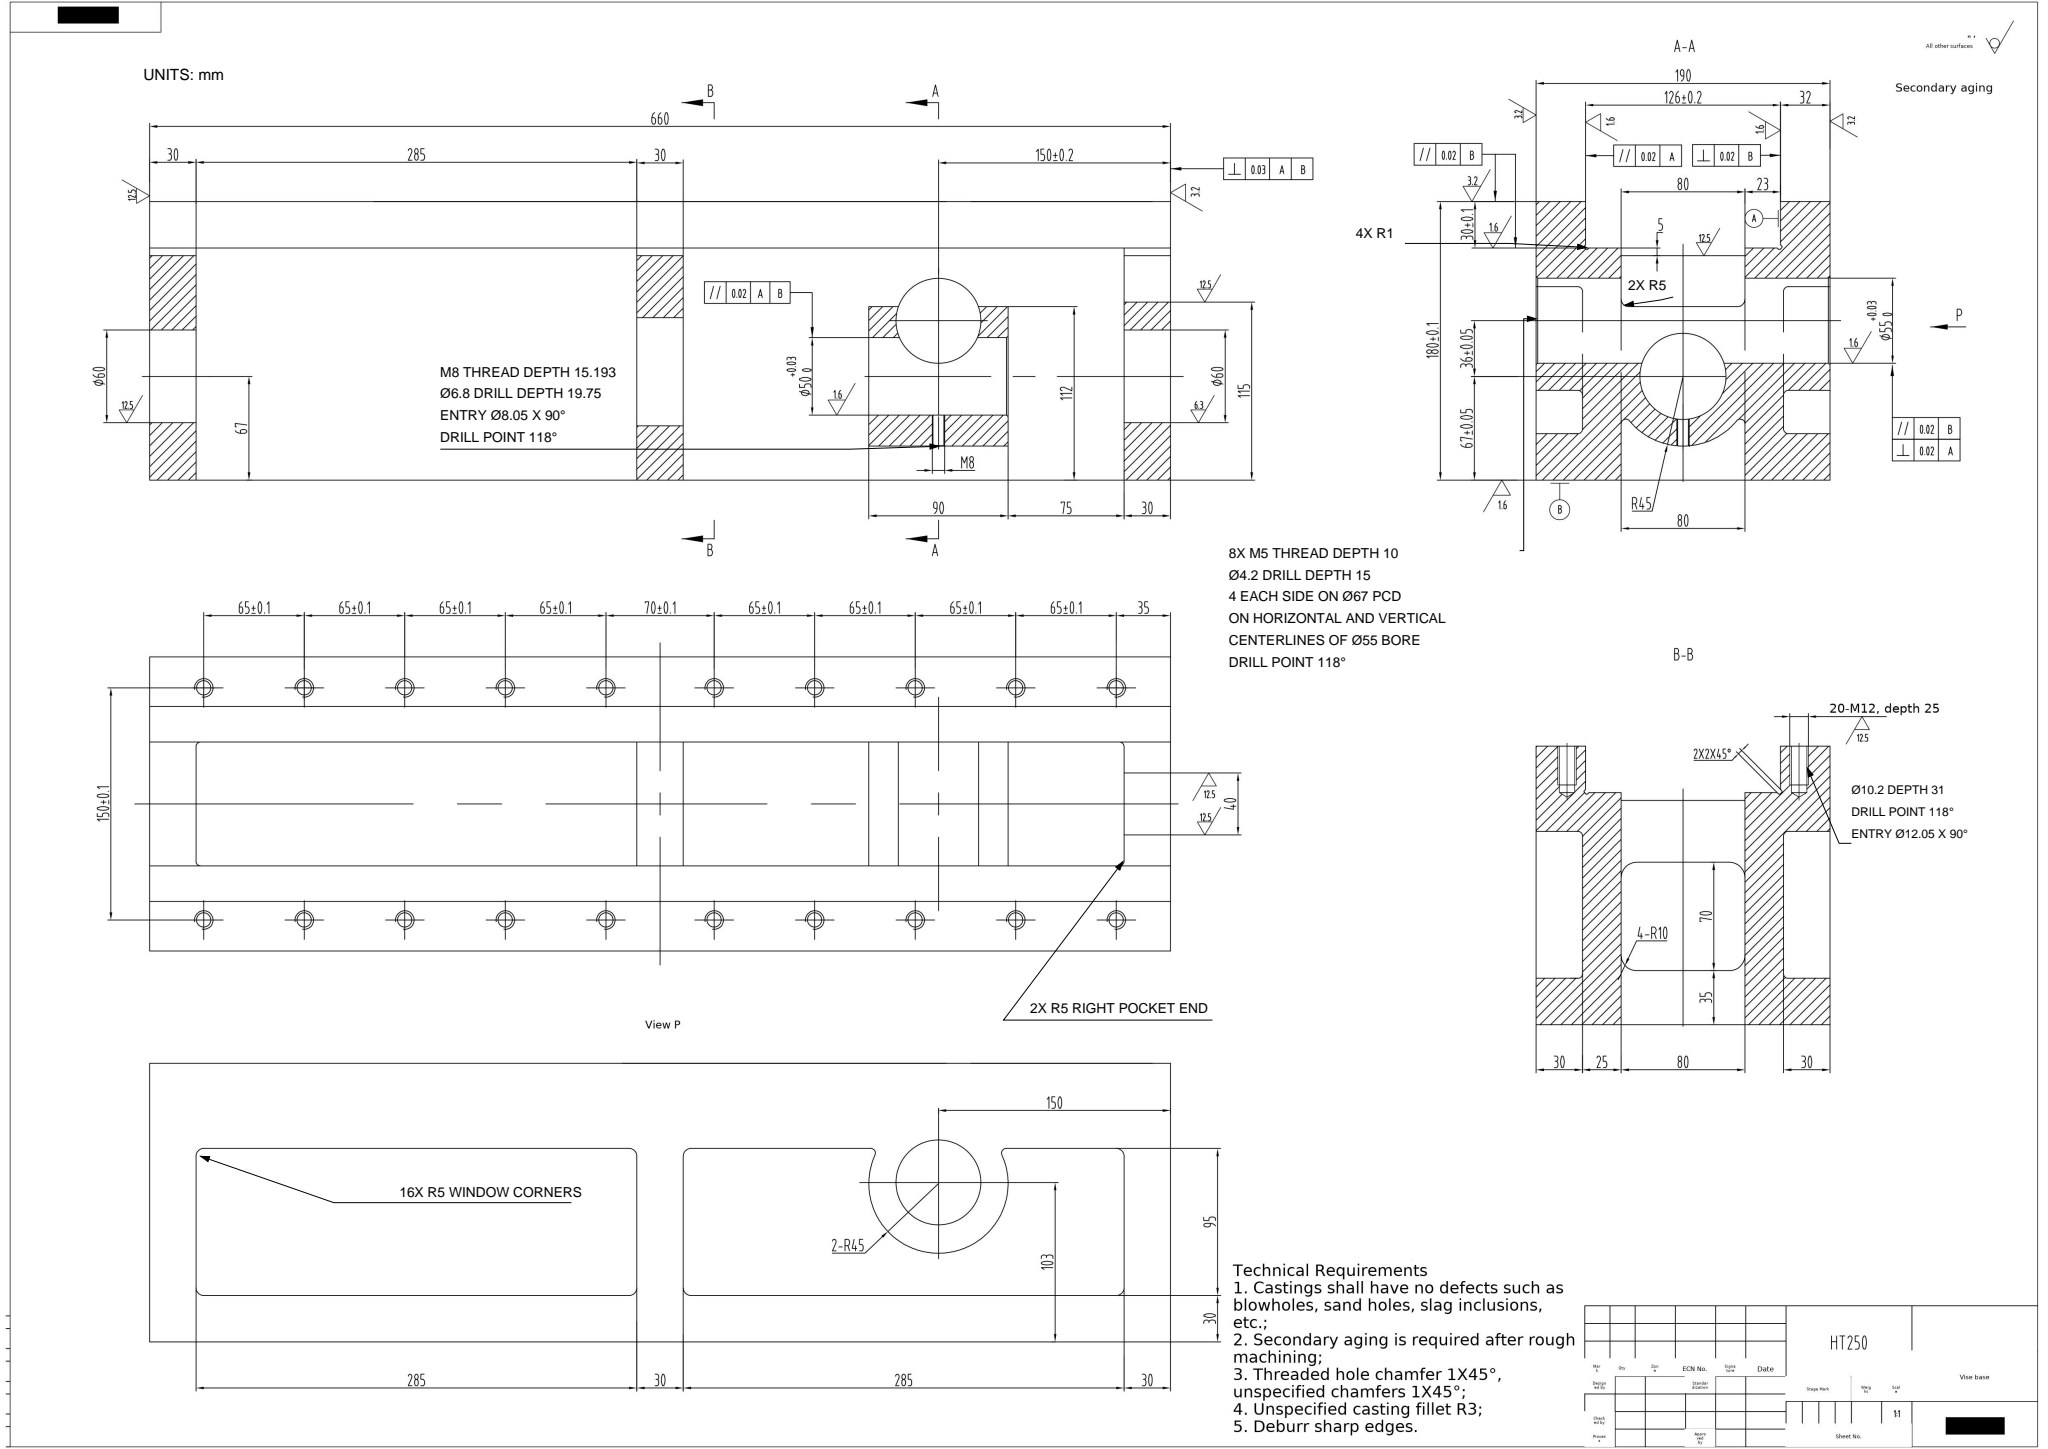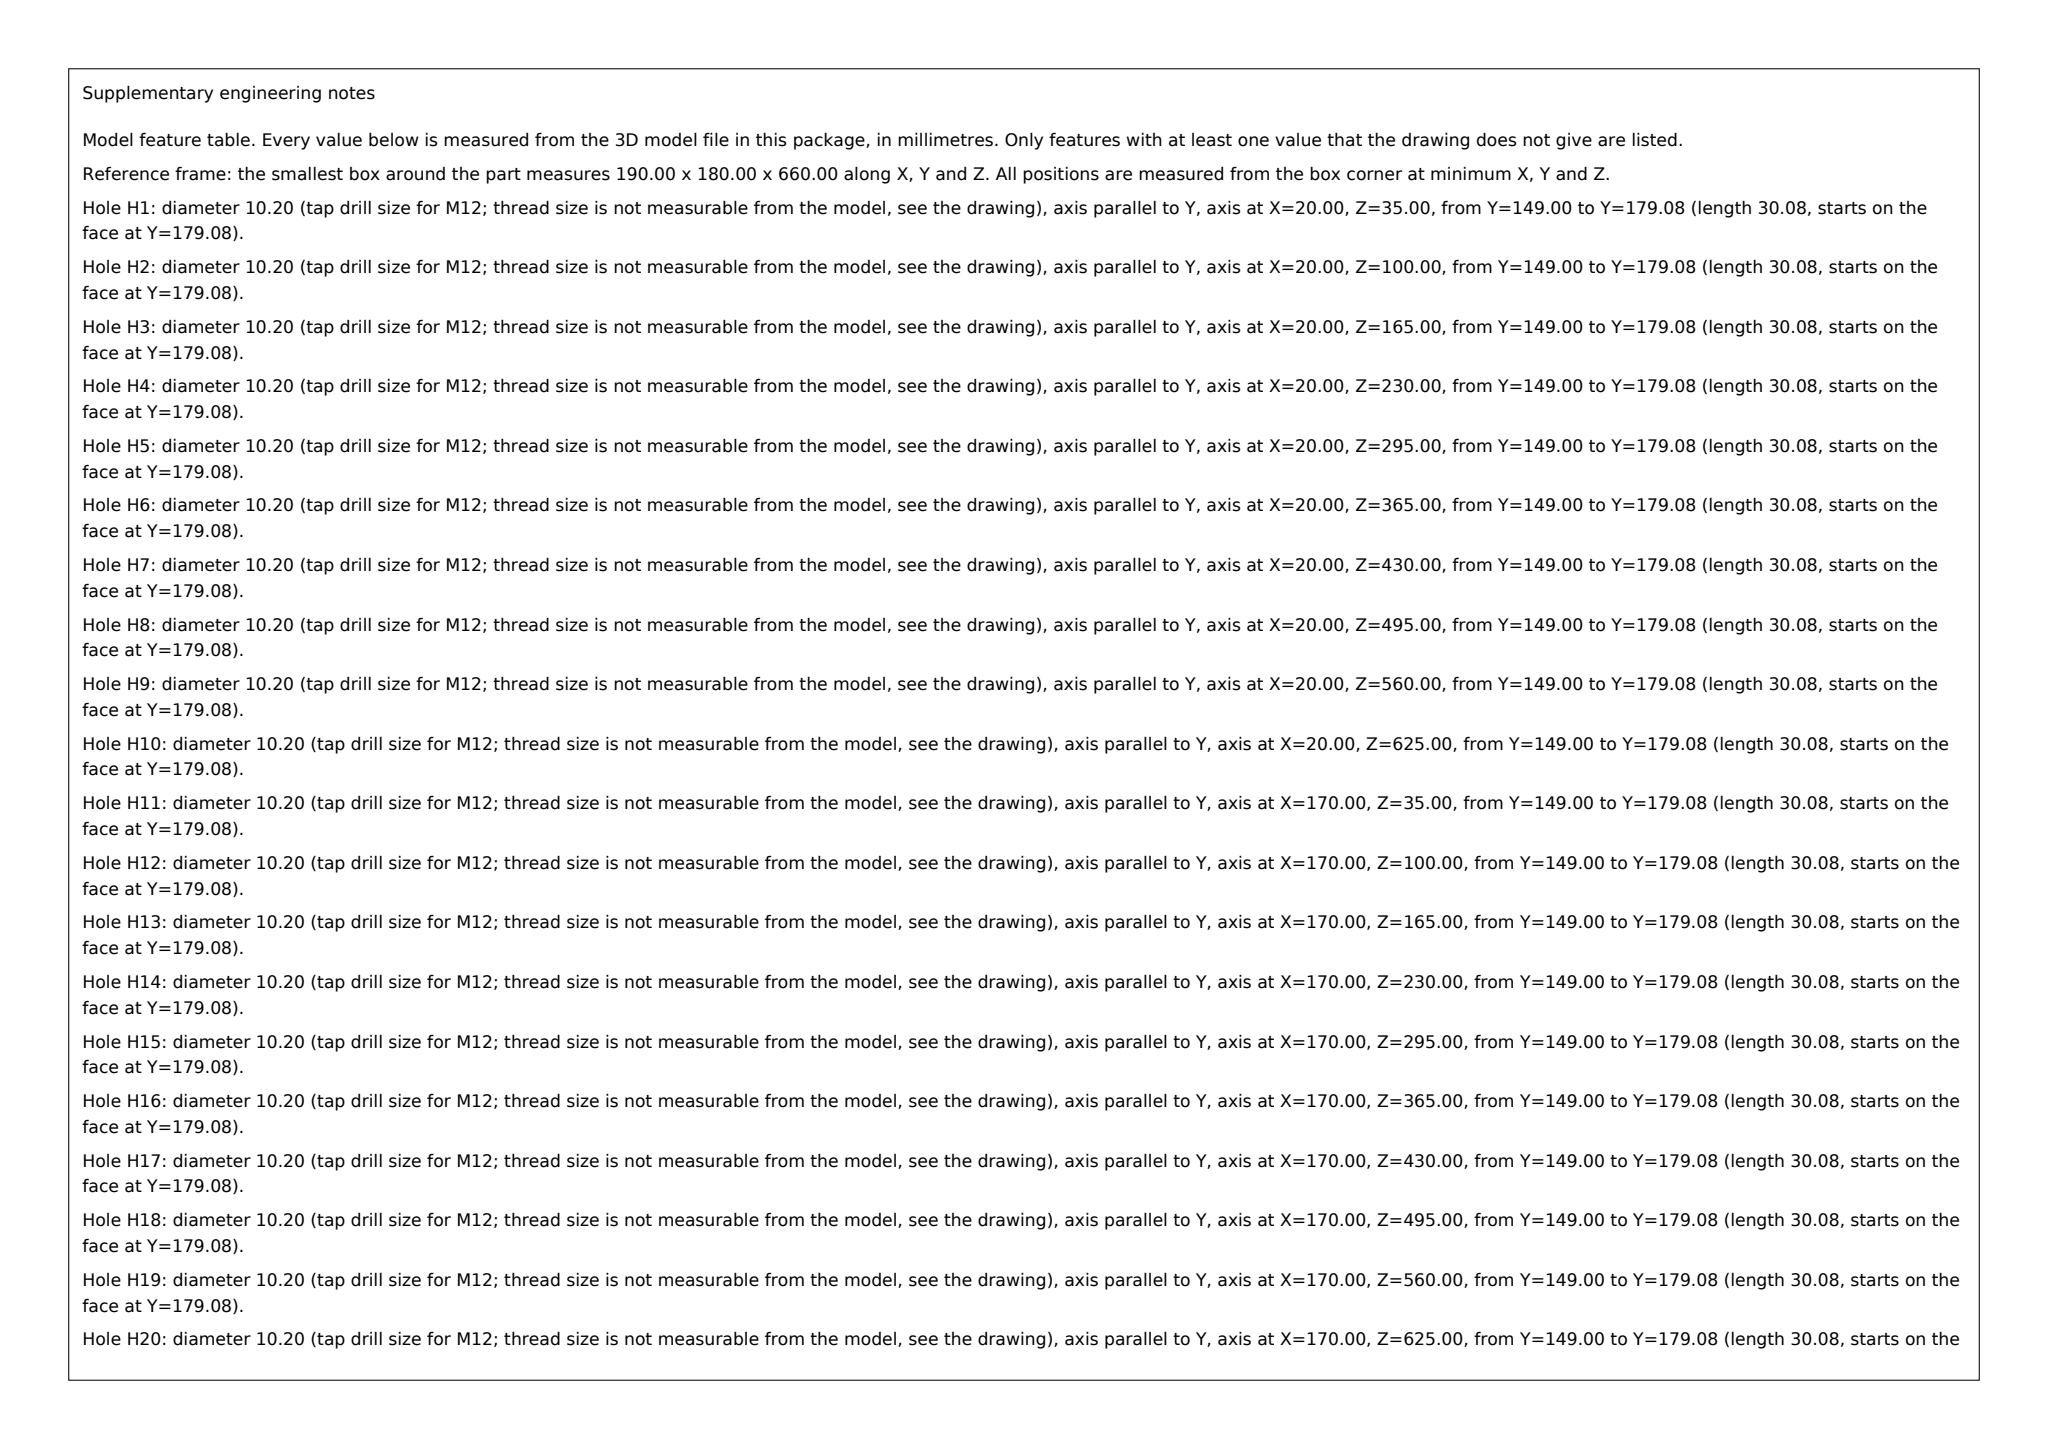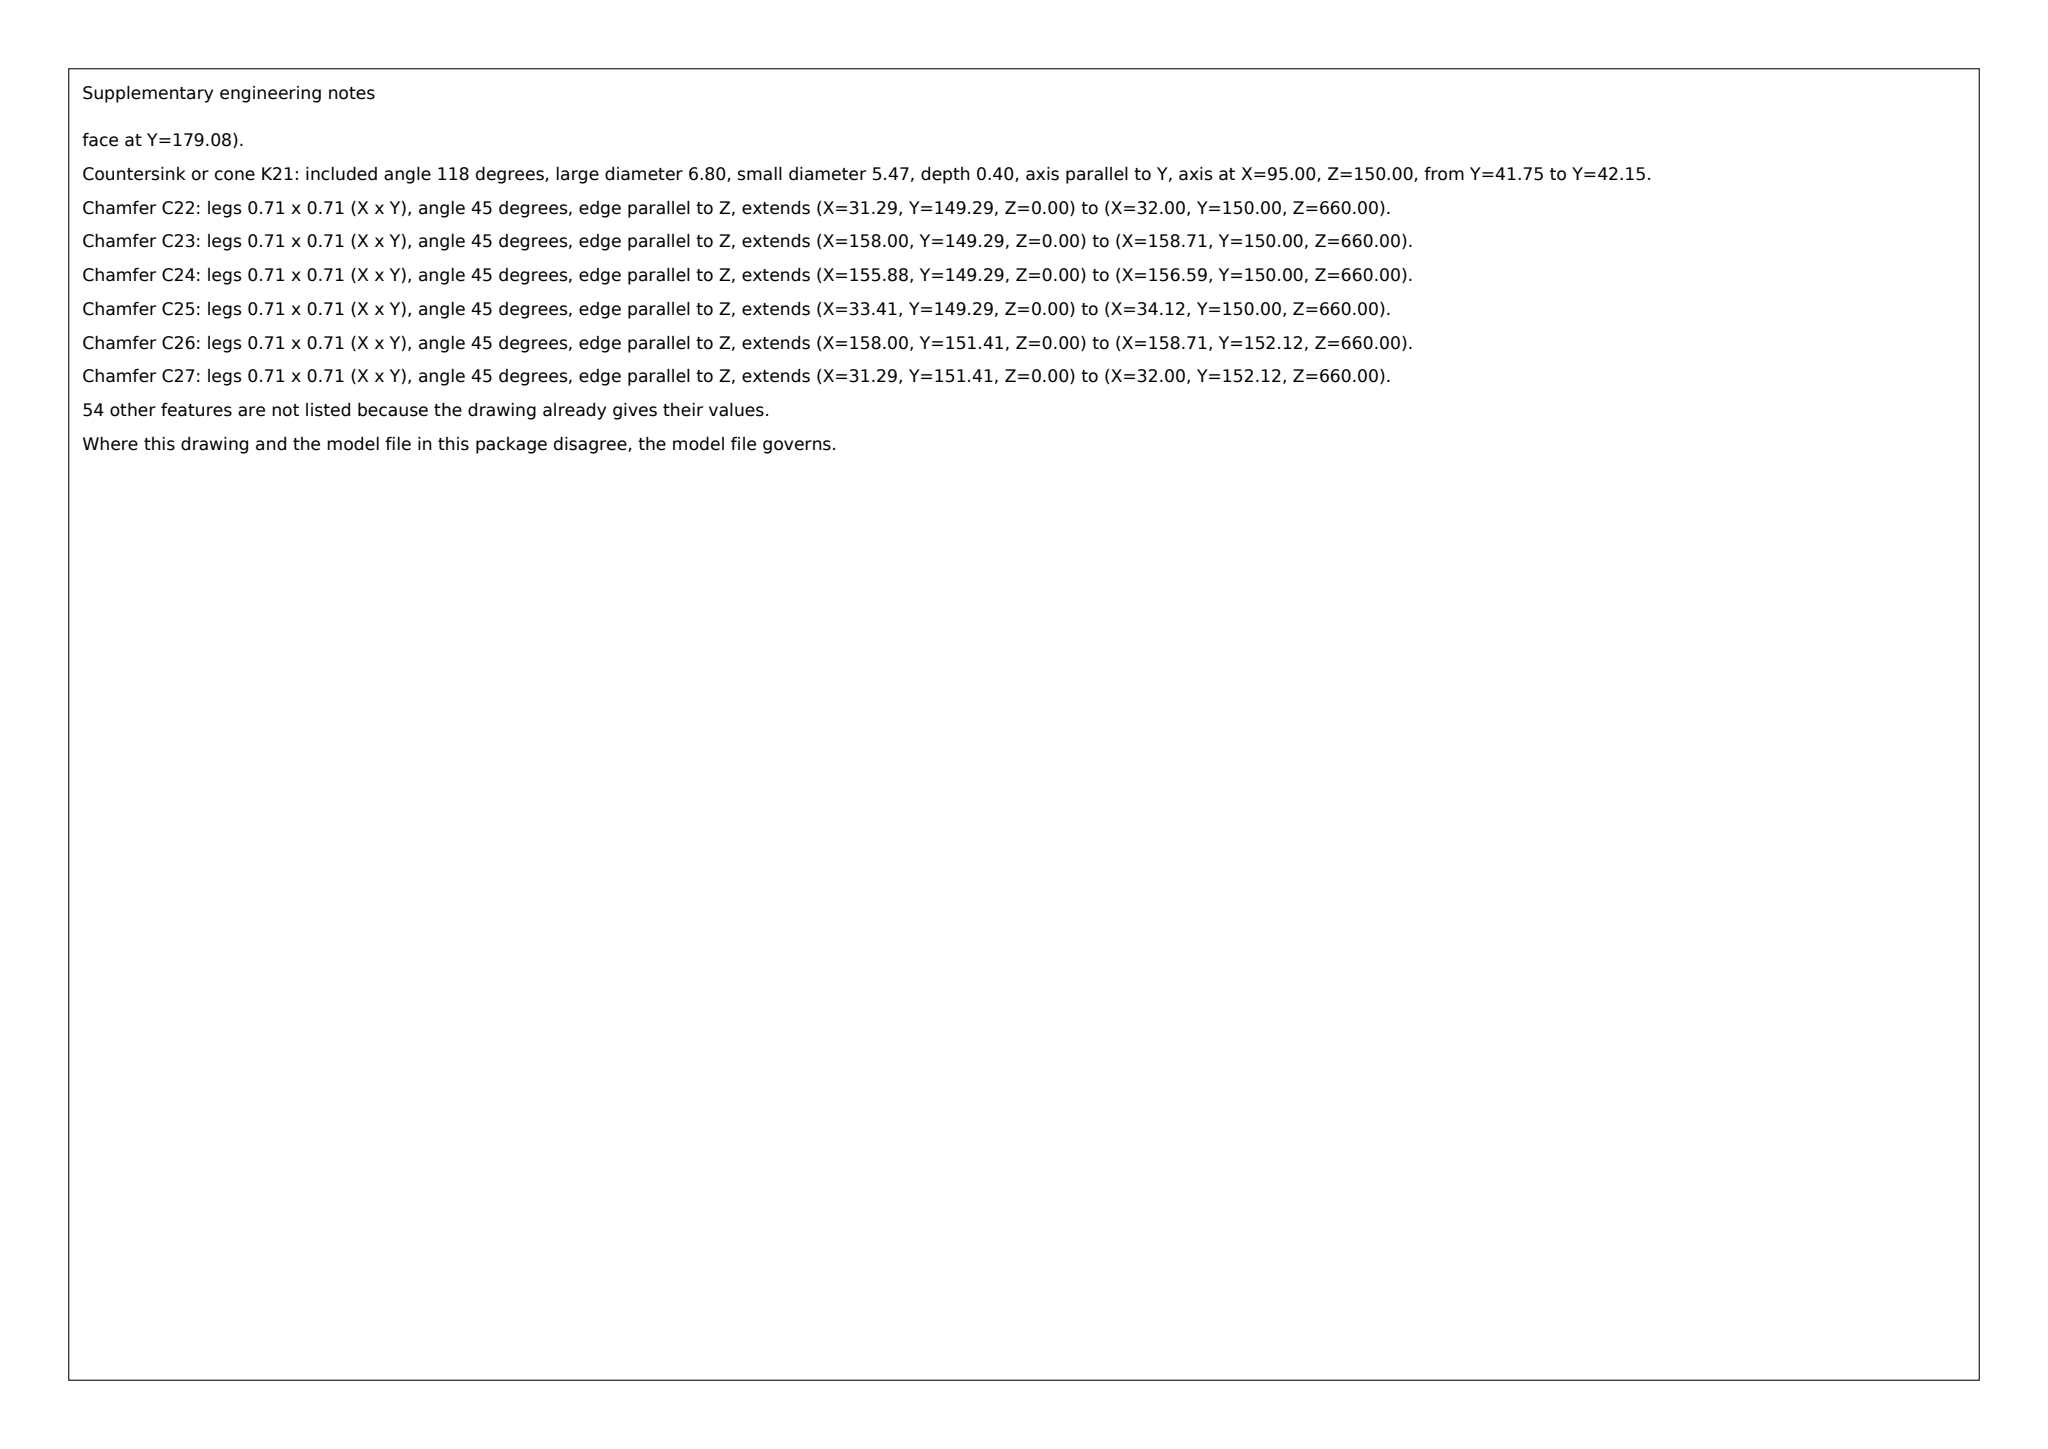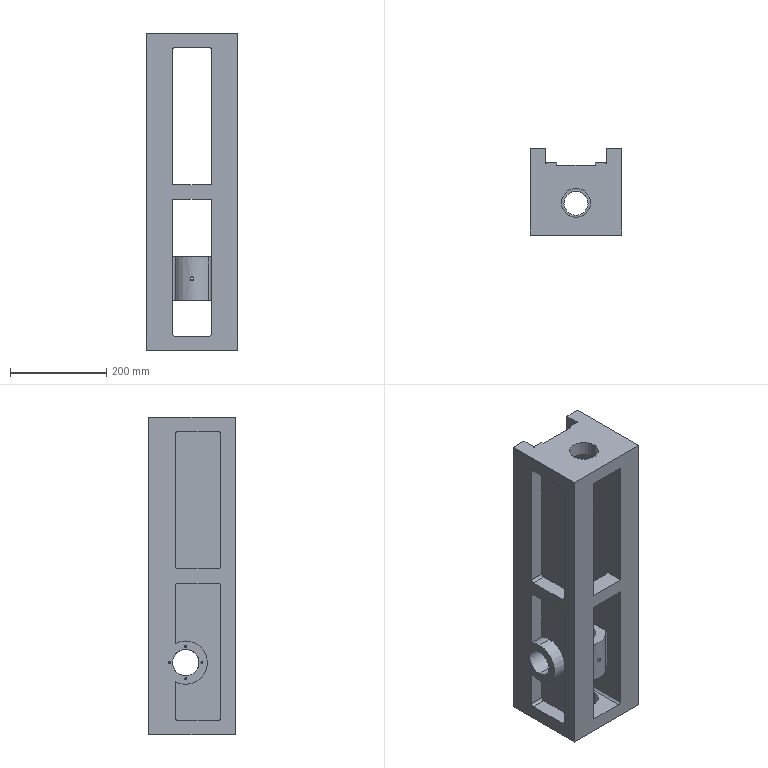Part | SolidWorks | mm | material HT250 | 1 solid | 268 faces | box 190 x 180 x 660 mm | volume 9879127 mm3 | cylinder 108 | cone 100 | plane 60 | commonest cylinder face diameters 10.2 x40 10 x22 4.2 x16 90 x7 2 x5 60 x4 6 x4 20 x4